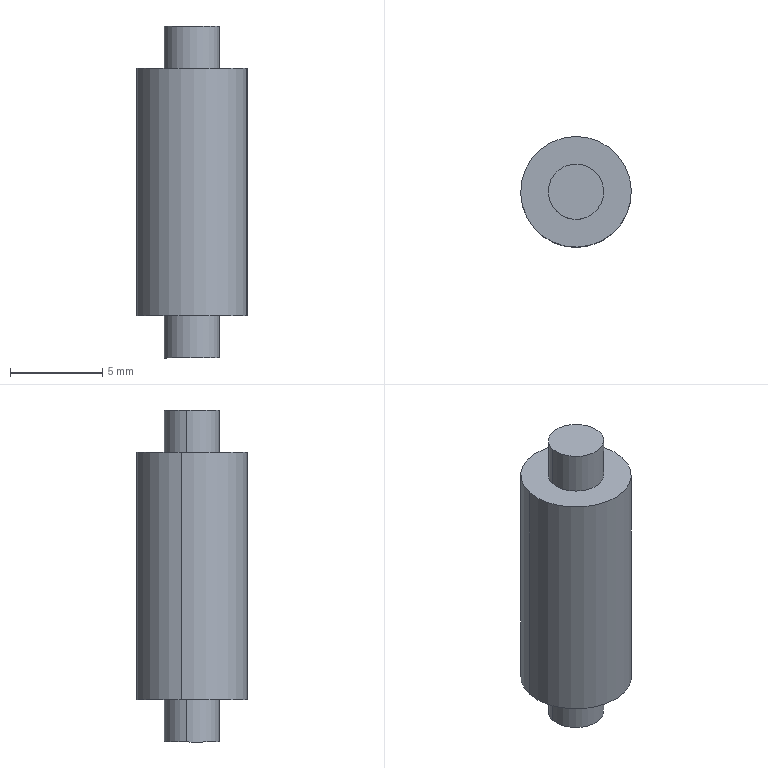Component | SolidWorks | Half-1_Axis-2 | 1 solid | 10 faces | box 6 x 6 x 18 mm | volume 411 mm3 | cylinder 6 | plane 4 | commonest cylinder face diameters 3 x4 6 x2 | material Copper
build123d program:
from build123d import *

# Parameters (mm, degrees)
SKETCH1_R           = 3
BOSS_EXTRUDE1_DEPTH = 6.7
SKETCH2_R           = 1.5
BOSS_EXTRUDE2_DEPTH = 2.3
BOSS_EXTRUDE3_START = 2.3
SKETCH3_R           = 1.5
BOSS_EXTRUDE3_DEPTH = 2.3


with BuildPart() as part:
    # Sketch1 → Boss-Extrude1 (new, symmetric)
    with BuildSketch(Plane.XY):
        Circle(SKETCH1_R)
    extrude(amount=BOSS_EXTRUDE1_DEPTH, both=True)

    # Sketch2 → Boss-Extrude2 (add)
    with BuildSketch(Plane.XY.offset(6.7)):
        Circle(SKETCH2_R)
    extrude(amount=BOSS_EXTRUDE2_DEPTH)

    # Sketch3 → Boss-Extrude3 (add)
    with BuildSketch(Plane(origin=(0, 0, -6.7), x_dir=(-1, 0, 0), z_dir=(0, 0, -1)).offset(BOSS_EXTRUDE3_START)):
        with Locations(Location((0, 0, 0), (0, 0, 180))):
            Circle(SKETCH3_R)
    extrude(amount=-BOSS_EXTRUDE3_DEPTH)


solid = part.part

# Placed as in the assembly
solid = solid.moved(Location((-19.269, -2.1, 37), (0, 0, 0)))
STEP:
#1=COLOUR_RGB('',0.7922,0.8196,0.9333);
#2=FILL_AREA_STYLE_COLOUR('',#1);
#3=FILL_AREA_STYLE('',(#2));
#4=SURFACE_STYLE_FILL_AREA(#3);
#5=SURFACE_SIDE_STYLE('',(#4));
#6=SURFACE_STYLE_USAGE(.BOTH.,#5);
#7=PRESENTATION_STYLE_ASSIGNMENT((#6));
#8=CARTESIAN_POINT('',(-0.8165,-0.07116,1.102));
#9=VERTEX_POINT('',#8);
#10=CARTESIAN_POINT('',(-0.7007,-0.09422,1.102));
#11=VERTEX_POINT('',#10);
#12=CARTESIAN_POINT('',(-0.7586,-0.08269,1.102));
#13=DIRECTION('',(0.,0.,-1.));
#14=DIRECTION('',(-0.9807,0.1953,-0.));
#15=AXIS2_PLACEMENT_3D('',#12,#13,#14);
#16=CIRCLE('',#15,0.05906);
#17=EDGE_CURVE('',#9,#11,#16,.T.);
#18=ORIENTED_EDGE('',*,*,#17,.F.);
#19=CARTESIAN_POINT('',(-0.8165,-0.07116,1.193));
#20=VERTEX_POINT('',#19);
#21=CARTESIAN_POINT('',(-0.8165,-0.07116,1.102));
#22=DIRECTION('',(-0.,-0.,1.));
#23=VECTOR('',#22,39.37);
#24=LINE('',#21,#23);
#25=EDGE_CURVE('',#9,#20,#24,.T.);
#26=ORIENTED_EDGE('',*,*,#25,.T.);
#27=CARTESIAN_POINT('',(-0.7007,-0.09422,1.193));
#28=VERTEX_POINT('',#27);
#29=CARTESIAN_POINT('',(-0.7586,-0.08269,1.193));
#30=DIRECTION('',(0.,0.,-1.));
#31=DIRECTION('',(0.9807,-0.1953,0.));
#32=AXIS2_PLACEMENT_3D('',#29,#30,#31);
#33=CIRCLE('',#32,0.05906);
#34=EDGE_CURVE('',#20,#28,#33,.T.);
#35=ORIENTED_EDGE('',*,*,#34,.T.);
#36=CARTESIAN_POINT('',(-0.7007,-0.09422,1.102));
#37=DIRECTION('',(-0.,-0.,1.));
#38=VECTOR('',#37,39.37);
#39=LINE('',#36,#38);
#40=EDGE_CURVE('',#11,#28,#39,.T.);
#41=ORIENTED_EDGE('',*,*,#40,.F.);
#42=EDGE_LOOP('',(#18,#26,#35,#41));
#43=FACE_OUTER_BOUND('',#42,.T.);
#44=CARTESIAN_POINT('',(-0.7586,-0.08269,1.102));
#45=DIRECTION('',(-0.,-0.,1.));
#46=DIRECTION('',(0.9807,-0.1953,0.));
#47=AXIS2_PLACEMENT_3D('',#44,#45,#46);
#48=CYLINDRICAL_SURFACE('',#47,0.05906);
#49=ADVANCED_FACE('',(#43),#48,.T.);
#50=CARTESIAN_POINT('',(-0.7007,-0.09422,1.811));
#51=VERTEX_POINT('',#50);
#52=CARTESIAN_POINT('',(-0.8165,-0.07116,1.811));
#53=VERTEX_POINT('',#52);
#54=CARTESIAN_POINT('',(-0.7586,-0.08269,1.811));
#55=DIRECTION('',(-0.,-0.,1.));
#56=DIRECTION('',(0.9807,-0.1953,0.));
#57=AXIS2_PLACEMENT_3D('',#54,#55,#56);
#58=CIRCLE('',#57,0.05906);
#59=EDGE_CURVE('',#51,#53,#58,.T.);
#60=ORIENTED_EDGE('',*,*,#59,.F.);
#61=CARTESIAN_POINT('',(-0.7007,-0.09422,1.72));
#62=VERTEX_POINT('',#61);
#63=CARTESIAN_POINT('',(-0.7007,-0.09422,1.811));
#64=DIRECTION('',(0.,0.,-1.));
#65=VECTOR('',#64,39.37);
#66=LINE('',#63,#65);
#67=EDGE_CURVE('',#51,#62,#66,.T.);
#68=ORIENTED_EDGE('',*,*,#67,.T.);
#69=CARTESIAN_POINT('',(-0.8165,-0.07116,1.72));
#70=VERTEX_POINT('',#69);
#71=CARTESIAN_POINT('',(-0.7586,-0.08269,1.72));
#72=DIRECTION('',(-0.,-0.,1.));
#73=DIRECTION('',(0.9807,-0.1953,0.));
#74=AXIS2_PLACEMENT_3D('',#71,#72,#73);
#75=CIRCLE('',#74,0.05906);
#76=EDGE_CURVE('',#62,#70,#75,.T.);
#77=ORIENTED_EDGE('',*,*,#76,.T.);
#78=CARTESIAN_POINT('',(-0.8165,-0.07116,1.811));
#79=DIRECTION('',(0.,0.,-1.));
#80=VECTOR('',#79,39.37);
#81=LINE('',#78,#80);
#82=EDGE_CURVE('',#53,#70,#81,.T.);
#83=ORIENTED_EDGE('',*,*,#82,.F.);
#84=EDGE_LOOP('',(#60,#68,#77,#83));
#85=FACE_OUTER_BOUND('',#84,.T.);
#86=CARTESIAN_POINT('',(-0.7586,-0.08269,1.811));
#87=DIRECTION('',(0.,0.,-1.));
#88=DIRECTION('',(-0.9807,0.1953,-0.));
#89=AXIS2_PLACEMENT_3D('',#86,#87,#88);
#90=CYLINDRICAL_SURFACE('',#89,0.05906);
#91=ADVANCED_FACE('',(#85),#90,.T.);
#92=CARTESIAN_POINT('',(-0.6428,-0.1058,1.72));
#93=VERTEX_POINT('',#92);
#94=CARTESIAN_POINT('',(-0.8745,-0.05962,1.72));
#95=VERTEX_POINT('',#94);
#96=CARTESIAN_POINT('',(-0.7586,-0.08269,1.72));
#97=DIRECTION('',(-0.,-0.,1.));
#98=DIRECTION('',(0.9807,-0.1953,0.));
#99=AXIS2_PLACEMENT_3D('',#96,#97,#98);
#100=CIRCLE('',#99,0.1181);
#101=EDGE_CURVE('',#93,#95,#100,.T.);
#102=ORIENTED_EDGE('',*,*,#101,.F.);
#103=CARTESIAN_POINT('',(-0.6428,-0.1058,1.193));
#104=VERTEX_POINT('',#103);
#105=CARTESIAN_POINT('',(-0.6428,-0.1058,1.72));
#106=DIRECTION('',(0.,0.,-1.));
#107=VECTOR('',#106,39.37);
#108=LINE('',#105,#107);
#109=EDGE_CURVE('',#93,#104,#108,.T.);
#110=ORIENTED_EDGE('',*,*,#109,.T.);
#111=CARTESIAN_POINT('',(-0.8745,-0.05962,1.193));
#112=VERTEX_POINT('',#111);
#113=CARTESIAN_POINT('',(-0.7586,-0.08269,1.193));
#114=DIRECTION('',(-0.,-0.,1.));
#115=DIRECTION('',(0.9807,-0.1953,0.));
#116=AXIS2_PLACEMENT_3D('',#113,#114,#115);
#117=CIRCLE('',#116,0.1181);
#118=EDGE_CURVE('',#104,#112,#117,.T.);
#119=ORIENTED_EDGE('',*,*,#118,.T.);
#120=CARTESIAN_POINT('',(-0.8745,-0.05962,1.72));
#121=DIRECTION('',(0.,0.,-1.));
#122=VECTOR('',#121,39.37);
#123=LINE('',#120,#122);
#124=EDGE_CURVE('',#95,#112,#123,.T.);
#125=ORIENTED_EDGE('',*,*,#124,.F.);
#126=EDGE_LOOP('',(#102,#110,#119,#125));
#127=FACE_OUTER_BOUND('',#126,.T.);
#128=CARTESIAN_POINT('',(-0.7586,-0.08269,1.72));
#129=DIRECTION('',(0.,0.,-1.));
#130=DIRECTION('',(-0.9807,0.1953,-0.));
#131=AXIS2_PLACEMENT_3D('',#128,#129,#130);
#132=CYLINDRICAL_SURFACE('',#131,0.1181);
#133=ADVANCED_FACE('',(#127),#132,.T.);
#134=CARTESIAN_POINT('',(-0.7586,-0.08269,1.193));
#135=DIRECTION('',(-0.,-0.,1.));
#136=DIRECTION('',(0.9807,-0.1953,0.));
#137=AXIS2_PLACEMENT_3D('',#134,#135,#136);
#138=CIRCLE('',#137,0.1181);
#139=EDGE_CURVE('',#112,#104,#138,.T.);
#140=ORIENTED_EDGE('',*,*,#139,.F.);
#141=ORIENTED_EDGE('',*,*,#118,.F.);
#142=EDGE_LOOP('',(#140,#141));
#143=FACE_OUTER_BOUND('',#142,.T.);
#144=CARTESIAN_POINT('',(-0.7586,-0.08269,1.193));
#145=DIRECTION('',(0.,0.,-1.));
#146=DIRECTION('',(0.9807,-0.1953,0.));
#147=AXIS2_PLACEMENT_3D('',#144,#145,#146);
#148=CIRCLE('',#147,0.05906);
#149=EDGE_CURVE('',#28,#20,#148,.T.);
#150=ORIENTED_EDGE('',*,*,#149,.F.);
#151=ORIENTED_EDGE('',*,*,#34,.F.);
#152=EDGE_LOOP('',(#150,#151));
#153=FACE_BOUND('',#152,.T.);
#154=CARTESIAN_POINT('',(-0.7586,-0.08269,1.193));
#155=DIRECTION('',(-0.,-0.,1.));
#156=DIRECTION('',(0.9807,-0.1953,0.));
#157=AXIS2_PLACEMENT_3D('',#154,#155,#156);
#158=PLANE('',#157);
#159=ADVANCED_FACE('',(#143,#153),#158,.F.);
#160=CARTESIAN_POINT('',(-0.7586,-0.08269,1.72));
#161=DIRECTION('',(-0.,-0.,1.));
#162=DIRECTION('',(0.9807,-0.1953,0.));
#163=AXIS2_PLACEMENT_3D('',#160,#161,#162);
#164=CIRCLE('',#163,0.1181);
#165=EDGE_CURVE('',#95,#93,#164,.T.);
#166=ORIENTED_EDGE('',*,*,#165,.T.);
#167=ORIENTED_EDGE('',*,*,#101,.T.);
#168=EDGE_LOOP('',(#166,#167));
#169=FACE_OUTER_BOUND('',#168,.T.);
#170=CARTESIAN_POINT('',(-0.7586,-0.08269,1.72));
#171=DIRECTION('',(-0.,-0.,1.));
#172=DIRECTION('',(0.9807,-0.1953,0.));
#173=AXIS2_PLACEMENT_3D('',#170,#171,#172);
#174=CIRCLE('',#173,0.05906);
#175=EDGE_CURVE('',#70,#62,#174,.T.);
#176=ORIENTED_EDGE('',*,*,#175,.F.);
#177=ORIENTED_EDGE('',*,*,#76,.F.);
#178=EDGE_LOOP('',(#176,#177));
#179=FACE_BOUND('',#178,.T.);
#180=CARTESIAN_POINT('',(-0.7586,-0.08269,1.72));
#181=DIRECTION('',(-0.,-0.,1.));
#182=DIRECTION('',(0.9807,-0.1953,0.));
#183=AXIS2_PLACEMENT_3D('',#180,#181,#182);
#184=PLANE('',#183);
#185=ADVANCED_FACE('',(#169,#179),#184,.T.);
#186=ORIENTED_EDGE('',*,*,#109,.F.);
#187=ORIENTED_EDGE('',*,*,#165,.F.);
#188=ORIENTED_EDGE('',*,*,#124,.T.);
#189=ORIENTED_EDGE('',*,*,#139,.T.);
#190=EDGE_LOOP('',(#186,#187,#188,#189));
#191=FACE_OUTER_BOUND('',#190,.T.);
#192=CARTESIAN_POINT('',(-0.7586,-0.08269,1.72));
#193=DIRECTION('',(0.,0.,-1.));
#194=DIRECTION('',(-0.9807,0.1953,-0.));
#195=AXIS2_PLACEMENT_3D('',#192,#193,#194);
#196=CYLINDRICAL_SURFACE('',#195,0.1181);
#197=ADVANCED_FACE('',(#191),#196,.T.);
#198=ORIENTED_EDGE('',*,*,#67,.F.);
#199=CARTESIAN_POINT('',(-0.7586,-0.08269,1.811));
#200=DIRECTION('',(-0.,-0.,1.));
#201=DIRECTION('',(0.9807,-0.1953,0.));
#202=AXIS2_PLACEMENT_3D('',#199,#200,#201);
#203=CIRCLE('',#202,0.05906);
#204=EDGE_CURVE('',#53,#51,#203,.T.);
#205=ORIENTED_EDGE('',*,*,#204,.F.);
#206=ORIENTED_EDGE('',*,*,#82,.T.);
#207=ORIENTED_EDGE('',*,*,#175,.T.);
#208=EDGE_LOOP('',(#198,#205,#206,#207));
#209=FACE_OUTER_BOUND('',#208,.T.);
#210=CARTESIAN_POINT('',(-0.7586,-0.08269,1.811));
#211=DIRECTION('',(0.,0.,-1.));
#212=DIRECTION('',(-0.9807,0.1953,-0.));
#213=AXIS2_PLACEMENT_3D('',#210,#211,#212);
#214=CYLINDRICAL_SURFACE('',#213,0.05906);
#215=ADVANCED_FACE('',(#209),#214,.T.);
#216=ORIENTED_EDGE('',*,*,#204,.T.);
#217=ORIENTED_EDGE('',*,*,#59,.T.);
#218=EDGE_LOOP('',(#216,#217));
#219=FACE_OUTER_BOUND('',#218,.T.);
#220=CARTESIAN_POINT('',(-0.7586,-0.08269,1.811));
#221=DIRECTION('',(-0.,-0.,1.));
#222=DIRECTION('',(0.9807,-0.1953,0.));
#223=AXIS2_PLACEMENT_3D('',#220,#221,#222);
#224=PLANE('',#223);
#225=ADVANCED_FACE('',(#219),#224,.T.);
#226=ORIENTED_EDGE('',*,*,#25,.F.);
#227=CARTESIAN_POINT('',(-0.7586,-0.08269,1.102));
#228=DIRECTION('',(0.,0.,-1.));
#229=DIRECTION('',(-0.9807,0.1953,-0.));
#230=AXIS2_PLACEMENT_3D('',#227,#228,#229);
#231=CIRCLE('',#230,0.05906);
#232=EDGE_CURVE('',#11,#9,#231,.T.);
#233=ORIENTED_EDGE('',*,*,#232,.F.);
#234=ORIENTED_EDGE('',*,*,#40,.T.);
#235=ORIENTED_EDGE('',*,*,#149,.T.);
#236=EDGE_LOOP('',(#226,#233,#234,#235));
#237=FACE_OUTER_BOUND('',#236,.T.);
#238=CARTESIAN_POINT('',(-0.7586,-0.08269,1.102));
#239=DIRECTION('',(-0.,-0.,1.));
#240=DIRECTION('',(0.9807,-0.1953,0.));
#241=AXIS2_PLACEMENT_3D('',#238,#239,#240);
#242=CYLINDRICAL_SURFACE('',#241,0.05906);
#243=ADVANCED_FACE('',(#237),#242,.T.);
#244=ORIENTED_EDGE('',*,*,#232,.T.);
#245=ORIENTED_EDGE('',*,*,#17,.T.);
#246=EDGE_LOOP('',(#244,#245));
#247=FACE_OUTER_BOUND('',#246,.T.);
#248=CARTESIAN_POINT('',(-0.7586,-0.08269,1.102));
#249=DIRECTION('',(0.,0.,-1.));
#250=DIRECTION('',(-0.9807,0.1953,-0.));
#251=AXIS2_PLACEMENT_3D('',#248,#249,#250);
#252=PLANE('',#251);
#253=ADVANCED_FACE('',(#247),#252,.T.);
#254=CLOSED_SHELL('',(#49,#91,#133,#159,#185,#197,#215,#225,#243,#253));
#255=MANIFOLD_SOLID_BREP('',#254);
#256=STYLED_ITEM('',(#7),#255);
#257=PRESENTATION_LAYER_ASSIGNMENT('','',(#256));
#258=CARTESIAN_POINT('',(0.,0.,0.));
#259=DIRECTION('',(0.,0.,1.));
#260=DIRECTION('',(1.,0.,0.));
#261=AXIS2_PLACEMENT_3D('',#258,#259,#260);
#262=(LENGTH_UNIT()NAMED_UNIT(*)SI_UNIT($,.METRE.));
#263=LENGTH_MEASURE_WITH_UNIT(LENGTH_MEASURE(0.0254),#262);
#264=DIMENSIONAL_EXPONENTS(1.,0.,0.,0.,0.,0.,0.);
#265=(CONVERSION_BASED_UNIT('',#263)LENGTH_UNIT()NAMED_UNIT(#264));
#266=UNCERTAINTY_MEASURE_WITH_UNIT(LENGTH_MEASURE(0.00001),#265,'','');
#267=(NAMED_UNIT(*)PLANE_ANGLE_UNIT()SI_UNIT($,.RADIAN.));
#268=(NAMED_UNIT(*)SI_UNIT($,.STERADIAN.)SOLID_ANGLE_UNIT());
#269=(GEOMETRIC_REPRESENTATION_CONTEXT(3)GLOBAL_UNCERTAINTY_ASSIGNED_CONTEXT((#266))GLOBAL_UNIT_ASSIGNED_CONTEXT((#265,#267,#268))REPRESENTATION_CONTEXT('',''));
#270=ADVANCED_BREP_SHAPE_REPRESENTATION('',(#255,#261),#269);
#271=(LENGTH_UNIT()NAMED_UNIT(*)SI_UNIT($,.METRE.));
#272=LENGTH_MEASURE_WITH_UNIT(LENGTH_MEASURE(0.0254),#271);
#273=DIMENSIONAL_EXPONENTS(1.,0.,0.,0.,0.,0.,0.);
#274=(CONVERSION_BASED_UNIT('',#272)LENGTH_UNIT()NAMED_UNIT(#273));
#275=UNCERTAINTY_MEASURE_WITH_UNIT(LENGTH_MEASURE(0.00001),#274,'','');
#276=(NAMED_UNIT(*)PLANE_ANGLE_UNIT()SI_UNIT($,.RADIAN.));
#277=(NAMED_UNIT(*)SI_UNIT($,.STERADIAN.)SOLID_ANGLE_UNIT());
#278=(GEOMETRIC_REPRESENTATION_CONTEXT(3)GLOBAL_UNCERTAINTY_ASSIGNED_CONTEXT((#275))GLOBAL_UNIT_ASSIGNED_CONTEXT((#274,#276,#277))REPRESENTATION_CONTEXT('',''));
#279=MECHANICAL_DESIGN_GEOMETRIC_PRESENTATION_REPRESENTATION('',(#256),#278);